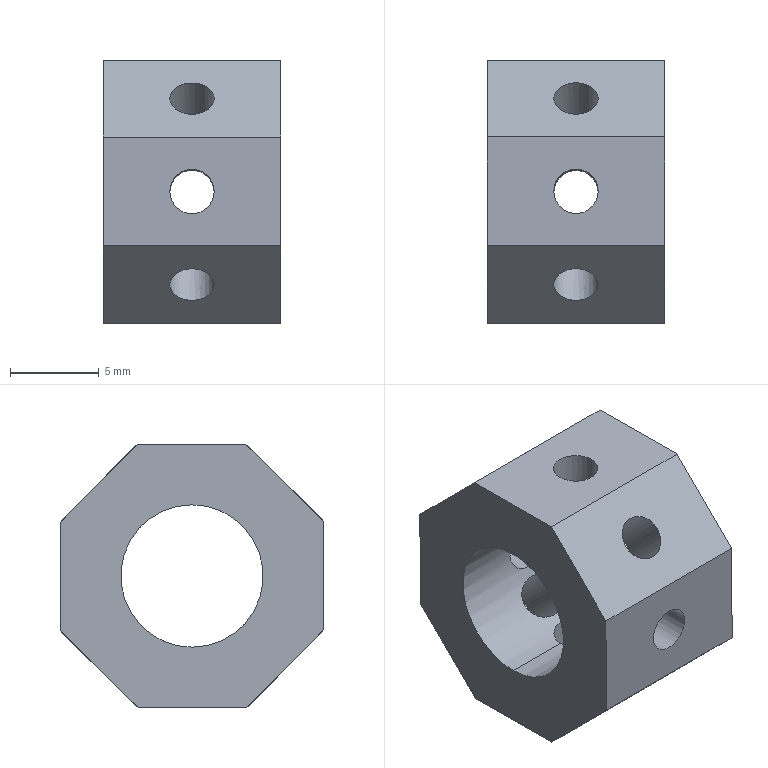Component | SolidWorks | Nut-1 | 1 solid | 28 faces | volume 1172 mm3 | cylinder 18 | plane 10 | commonest cylinder face diameters 2.5 x16 8 x2